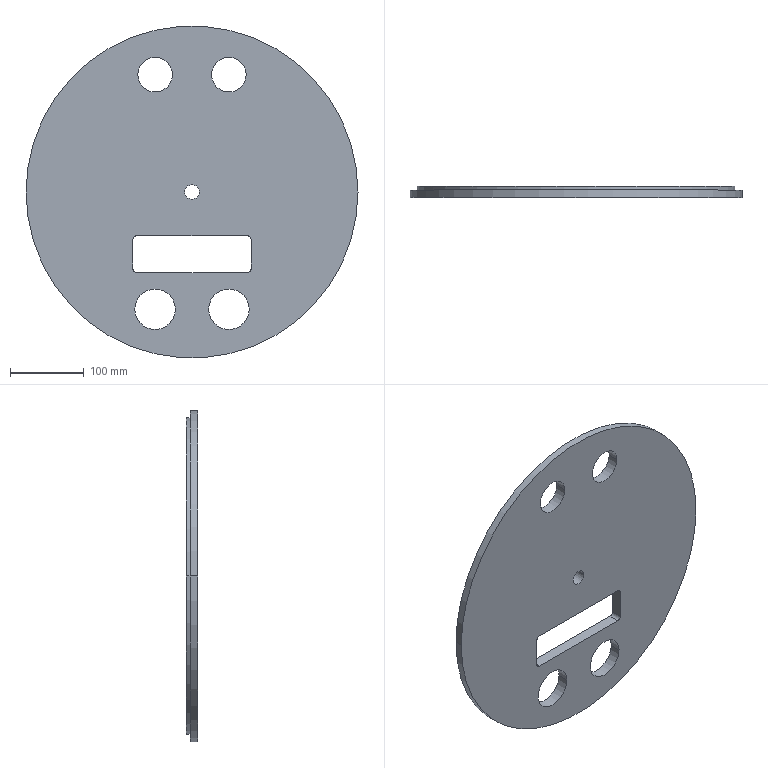Component | SolidWorks | Disc-1 | 1 solid | 25 faces | box 450 x 15 x 450 mm | volume 2068818 mm3 | cylinder 18 | plane 7 | commonest cylinder face diameters 47 x4 55 x4 10 x4 430 x2 20 x2 450 x2
build123d program:
from build123d import *

# Parameters (mm, degrees)
SKETCH1_R      = 225
EXTRUDE1_DEPTH = 15
SKETCH4_R      = 10
SKETCH4_R_2    = 27.5
SKETCH4_R_3    = 23.5
EXTRUDE3_DEPTH = 1808.804
EXTRUDE4_START = -5
SKETCH5_R      = 225
SKETCH5_R_2    = 215
EXTRUDE4_DEPTH = 5


with BuildPart() as part:
    # Sketch1 → Extrude1 (new body)
    with BuildSketch(Plane.XY):
        with Locations((1324.072, 706.83)):
            Circle(SKETCH1_R)
    extrude(amount=EXTRUDE1_DEPTH)

    # Sketch4 → Extrude3 (cut, through all)
    with BuildSketch(Plane(origin=(0, 0, 0), x_dir=(-1, 0, 0), z_dir=(0, 0, -1))):
        with Locations((-1324.072, 706.83)):
            Circle(SKETCH4_R)
        with Locations((-1374.072, 865.83)):
            Circle(SKETCH4_R_2)
        with Locations((-1274.072, 865.83)):
            Circle(SKETCH4_R_2)
        with Locations((-1374.072, 547.83)):
            Circle(SKETCH4_R_3)
        with Locations((-1274.072, 547.83)):
            Circle(SKETCH4_R_3)
        with BuildLine():
            Line((-1399.072, 766.33), (-1249.072, 766.33))
            ThreePointArc((-1249.072, 766.33), (-1245.536, 767.795), (-1244.072, 771.33))
            Line((-1244.072, 771.33), (-1244.072, 811.33))
            ThreePointArc((-1244.072, 811.33), (-1245.536, 814.866), (-1249.072, 816.33))
            Line((-1249.072, 816.33), (-1399.072, 816.33))
            ThreePointArc((-1399.072, 816.33), (-1402.607, 814.866), (-1404.072, 811.33))
            Line((-1404.072, 811.33), (-1404.072, 771.33))
            ThreePointArc((-1404.072, 771.33), (-1402.607, 767.795), (-1399.072, 766.33))
        make_face()
    extrude(amount=-EXTRUDE3_DEPTH, mode=Mode.SUBTRACT)

    # Sketch5 → Extrude4 (cut)
    with BuildSketch(Plane.XY.offset(15).offset(EXTRUDE4_START)):
        with Locations((1324.072, 706.83)):
            Circle(SKETCH5_R)
        with Locations((1324.072, 706.83)):
            Circle(SKETCH5_R_2, mode=Mode.SUBTRACT)
    extrude(amount=EXTRUDE4_DEPTH, mode=Mode.SUBTRACT)


solid = part.part

# Placed as in the assembly
solid = solid.moved(Location((-1488.855, 430.983, 710.83), (-90, 0, 0)))
STEP:
#1=COLOUR_RGB('',0.7922,0.8196,0.9333);
#2=FILL_AREA_STYLE_COLOUR('',#1);
#3=FILL_AREA_STYLE('',(#2));
#4=SURFACE_STYLE_FILL_AREA(#3);
#5=SURFACE_SIDE_STYLE('',(#4));
#6=SURFACE_STYLE_USAGE(.BOTH.,#5);
#7=PRESENTATION_STYLE_ASSIGNMENT((#6));
#8=CARTESIAN_POINT('',(1.977,17.362,0.1575));
#9=VERTEX_POINT('',#8);
#10=CARTESIAN_POINT('',(-14.952,17.362,0.1575));
#11=VERTEX_POINT('',#10);
#12=CARTESIAN_POINT('',(-6.488,17.362,0.1575));
#13=DIRECTION('',(0.,1.,0.));
#14=DIRECTION('',(1.,0.,-0.));
#15=AXIS2_PLACEMENT_3D('',#12,#13,#14);
#16=CIRCLE('',#15,8.465);
#17=EDGE_CURVE('',#9,#11,#16,.T.);
#18=ORIENTED_EDGE('',*,*,#17,.T.);
#19=CARTESIAN_POINT('',(-14.952,17.558,0.1575));
#20=VERTEX_POINT('',#19);
#21=CARTESIAN_POINT('',(-14.952,17.362,0.1575));
#22=DIRECTION('',(0.,1.,0.));
#23=VECTOR('',#22,39.37);
#24=LINE('',#21,#23);
#25=EDGE_CURVE('',#11,#20,#24,.T.);
#26=ORIENTED_EDGE('',*,*,#25,.T.);
#27=CARTESIAN_POINT('',(1.977,17.558,0.1575));
#28=VERTEX_POINT('',#27);
#29=CARTESIAN_POINT('',(-6.488,17.558,0.1575));
#30=DIRECTION('',(0.,1.,0.));
#31=DIRECTION('',(1.,0.,-0.));
#32=AXIS2_PLACEMENT_3D('',#29,#30,#31);
#33=CIRCLE('',#32,8.465);
#34=EDGE_CURVE('',#28,#20,#33,.T.);
#35=ORIENTED_EDGE('',*,*,#34,.F.);
#36=CARTESIAN_POINT('',(1.977,17.362,0.1575));
#37=DIRECTION('',(0.,1.,0.));
#38=VECTOR('',#37,39.37);
#39=LINE('',#36,#38);
#40=EDGE_CURVE('',#9,#28,#39,.T.);
#41=ORIENTED_EDGE('',*,*,#40,.F.);
#42=EDGE_LOOP('',(#18,#26,#35,#41));
#43=FACE_OUTER_BOUND('',#42,.T.);
#44=CARTESIAN_POINT('',(-6.488,17.362,0.1575));
#45=DIRECTION('',(0.,1.,0.));
#46=DIRECTION('',(1.,0.,-0.));
#47=AXIS2_PLACEMENT_3D('',#44,#45,#46);
#48=CYLINDRICAL_SURFACE('',#47,8.465);
#49=ADVANCED_FACE('',(#43),#48,.T.);
#50=CARTESIAN_POINT('',(-7.531,17.558,6.417));
#51=VERTEX_POINT('',#50);
#52=CARTESIAN_POINT('',(-9.381,17.558,6.417));
#53=VERTEX_POINT('',#52);
#54=CARTESIAN_POINT('',(-8.456,17.558,6.417));
#55=DIRECTION('',(0.,-1.,0.));
#56=DIRECTION('',(-1.,0.,0.));
#57=AXIS2_PLACEMENT_3D('',#54,#55,#56);
#58=CIRCLE('',#57,0.9252);
#59=EDGE_CURVE('',#51,#53,#58,.T.);
#60=ORIENTED_EDGE('',*,*,#59,.F.);
#61=CARTESIAN_POINT('',(-7.531,16.968,6.417));
#62=VERTEX_POINT('',#61);
#63=CARTESIAN_POINT('',(-7.531,17.558,6.417));
#64=DIRECTION('',(0.,-1.,0.));
#65=VECTOR('',#64,39.37);
#66=LINE('',#63,#65);
#67=EDGE_CURVE('',#51,#62,#66,.T.);
#68=ORIENTED_EDGE('',*,*,#67,.T.);
#69=CARTESIAN_POINT('',(-9.381,16.968,6.417));
#70=VERTEX_POINT('',#69);
#71=CARTESIAN_POINT('',(-8.456,16.968,6.417));
#72=DIRECTION('',(0.,-1.,0.));
#73=DIRECTION('',(-1.,0.,0.));
#74=AXIS2_PLACEMENT_3D('',#71,#72,#73);
#75=CIRCLE('',#74,0.9252);
#76=EDGE_CURVE('',#62,#70,#75,.T.);
#77=ORIENTED_EDGE('',*,*,#76,.T.);
#78=CARTESIAN_POINT('',(-9.381,17.558,6.417));
#79=DIRECTION('',(0.,-1.,0.));
#80=VECTOR('',#79,39.37);
#81=LINE('',#78,#80);
#82=EDGE_CURVE('',#53,#70,#81,.T.);
#83=ORIENTED_EDGE('',*,*,#82,.F.);
#84=EDGE_LOOP('',(#60,#68,#77,#83));
#85=FACE_OUTER_BOUND('',#84,.T.);
#86=CARTESIAN_POINT('',(-8.456,17.558,6.417));
#87=DIRECTION('',(0.,-1.,0.));
#88=DIRECTION('',(-1.,0.,0.));
#89=AXIS2_PLACEMENT_3D('',#86,#87,#88);
#90=CYLINDRICAL_SURFACE('',#89,0.9252);
#91=ADVANCED_FACE('',(#85),#90,.F.);
#92=CARTESIAN_POINT('',(-3.594,17.558,6.417));
#93=VERTEX_POINT('',#92);
#94=CARTESIAN_POINT('',(-5.444,17.558,6.417));
#95=VERTEX_POINT('',#94);
#96=CARTESIAN_POINT('',(-4.519,17.558,6.417));
#97=DIRECTION('',(0.,-1.,0.));
#98=DIRECTION('',(-1.,0.,0.));
#99=AXIS2_PLACEMENT_3D('',#96,#97,#98);
#100=CIRCLE('',#99,0.9252);
#101=EDGE_CURVE('',#93,#95,#100,.T.);
#102=ORIENTED_EDGE('',*,*,#101,.F.);
#103=CARTESIAN_POINT('',(-3.594,16.968,6.417));
#104=VERTEX_POINT('',#103);
#105=CARTESIAN_POINT('',(-3.594,17.558,6.417));
#106=DIRECTION('',(0.,-1.,0.));
#107=VECTOR('',#106,39.37);
#108=LINE('',#105,#107);
#109=EDGE_CURVE('',#93,#104,#108,.T.);
#110=ORIENTED_EDGE('',*,*,#109,.T.);
#111=CARTESIAN_POINT('',(-5.444,16.968,6.417));
#112=VERTEX_POINT('',#111);
#113=CARTESIAN_POINT('',(-4.519,16.968,6.417));
#114=DIRECTION('',(0.,-1.,0.));
#115=DIRECTION('',(-1.,0.,0.));
#116=AXIS2_PLACEMENT_3D('',#113,#114,#115);
#117=CIRCLE('',#116,0.9252);
#118=EDGE_CURVE('',#104,#112,#117,.T.);
#119=ORIENTED_EDGE('',*,*,#118,.T.);
#120=CARTESIAN_POINT('',(-5.444,17.558,6.417));
#121=DIRECTION('',(0.,-1.,0.));
#122=VECTOR('',#121,39.37);
#123=LINE('',#120,#122);
#124=EDGE_CURVE('',#95,#112,#123,.T.);
#125=ORIENTED_EDGE('',*,*,#124,.F.);
#126=EDGE_LOOP('',(#102,#110,#119,#125));
#127=FACE_OUTER_BOUND('',#126,.T.);
#128=CARTESIAN_POINT('',(-4.519,17.558,6.417));
#129=DIRECTION('',(0.,-1.,0.));
#130=DIRECTION('',(-1.,0.,0.));
#131=AXIS2_PLACEMENT_3D('',#128,#129,#130);
#132=CYLINDRICAL_SURFACE('',#131,0.9252);
#133=ADVANCED_FACE('',(#127),#132,.F.);
#134=CARTESIAN_POINT('',(-7.373,17.558,-6.102));
#135=VERTEX_POINT('',#134);
#136=CARTESIAN_POINT('',(-9.539,17.558,-6.102));
#137=VERTEX_POINT('',#136);
#138=CARTESIAN_POINT('',(-8.456,17.558,-6.102));
#139=DIRECTION('',(0.,-1.,0.));
#140=DIRECTION('',(-1.,0.,0.));
#141=AXIS2_PLACEMENT_3D('',#138,#139,#140);
#142=CIRCLE('',#141,1.083);
#143=EDGE_CURVE('',#135,#137,#142,.T.);
#144=ORIENTED_EDGE('',*,*,#143,.F.);
#145=CARTESIAN_POINT('',(-7.373,16.968,-6.102));
#146=VERTEX_POINT('',#145);
#147=CARTESIAN_POINT('',(-7.373,17.558,-6.102));
#148=DIRECTION('',(0.,-1.,0.));
#149=VECTOR('',#148,39.37);
#150=LINE('',#147,#149);
#151=EDGE_CURVE('',#135,#146,#150,.T.);
#152=ORIENTED_EDGE('',*,*,#151,.T.);
#153=CARTESIAN_POINT('',(-9.539,16.968,-6.102));
#154=VERTEX_POINT('',#153);
#155=CARTESIAN_POINT('',(-8.456,16.968,-6.102));
#156=DIRECTION('',(0.,-1.,0.));
#157=DIRECTION('',(-1.,0.,0.));
#158=AXIS2_PLACEMENT_3D('',#155,#156,#157);
#159=CIRCLE('',#158,1.083);
#160=EDGE_CURVE('',#146,#154,#159,.T.);
#161=ORIENTED_EDGE('',*,*,#160,.T.);
#162=CARTESIAN_POINT('',(-9.539,17.558,-6.102));
#163=DIRECTION('',(0.,-1.,0.));
#164=VECTOR('',#163,39.37);
#165=LINE('',#162,#164);
#166=EDGE_CURVE('',#137,#154,#165,.T.);
#167=ORIENTED_EDGE('',*,*,#166,.F.);
#168=EDGE_LOOP('',(#144,#152,#161,#167));
#169=FACE_OUTER_BOUND('',#168,.T.);
#170=CARTESIAN_POINT('',(-8.456,17.558,-6.102));
#171=DIRECTION('',(0.,-1.,0.));
#172=DIRECTION('',(-1.,0.,0.));
#173=AXIS2_PLACEMENT_3D('',#170,#171,#172);
#174=CYLINDRICAL_SURFACE('',#173,1.083);
#175=ADVANCED_FACE('',(#169),#174,.F.);
#176=CARTESIAN_POINT('',(-3.436,17.558,-6.102));
#177=VERTEX_POINT('',#176);
#178=CARTESIAN_POINT('',(-5.602,17.558,-6.102));
#179=VERTEX_POINT('',#178);
#180=CARTESIAN_POINT('',(-4.519,17.558,-6.102));
#181=DIRECTION('',(0.,-1.,0.));
#182=DIRECTION('',(-1.,0.,0.));
#183=AXIS2_PLACEMENT_3D('',#180,#181,#182);
#184=CIRCLE('',#183,1.083);
#185=EDGE_CURVE('',#177,#179,#184,.T.);
#186=ORIENTED_EDGE('',*,*,#185,.F.);
#187=CARTESIAN_POINT('',(-3.436,16.968,-6.102));
#188=VERTEX_POINT('',#187);
#189=CARTESIAN_POINT('',(-3.436,17.558,-6.102));
#190=DIRECTION('',(0.,-1.,0.));
#191=VECTOR('',#190,39.37);
#192=LINE('',#189,#191);
#193=EDGE_CURVE('',#177,#188,#192,.T.);
#194=ORIENTED_EDGE('',*,*,#193,.T.);
#195=CARTESIAN_POINT('',(-5.602,16.968,-6.102));
#196=VERTEX_POINT('',#195);
#197=CARTESIAN_POINT('',(-4.519,16.968,-6.102));
#198=DIRECTION('',(0.,-1.,0.));
#199=DIRECTION('',(-1.,0.,0.));
#200=AXIS2_PLACEMENT_3D('',#197,#198,#199);
#201=CIRCLE('',#200,1.083);
#202=EDGE_CURVE('',#188,#196,#201,.T.);
#203=ORIENTED_EDGE('',*,*,#202,.T.);
#204=CARTESIAN_POINT('',(-5.602,17.558,-6.102));
#205=DIRECTION('',(0.,-1.,0.));
#206=VECTOR('',#205,39.37);
#207=LINE('',#204,#206);
#208=EDGE_CURVE('',#179,#196,#207,.T.);
#209=ORIENTED_EDGE('',*,*,#208,.F.);
#210=EDGE_LOOP('',(#186,#194,#203,#209));
#211=FACE_OUTER_BOUND('',#210,.T.);
#212=CARTESIAN_POINT('',(-4.519,17.558,-6.102));
#213=DIRECTION('',(0.,-1.,0.));
#214=DIRECTION('',(-1.,0.,0.));
#215=AXIS2_PLACEMENT_3D('',#212,#213,#214);
#216=CYLINDRICAL_SURFACE('',#215,1.083);
#217=ADVANCED_FACE('',(#211),#216,.F.);
#218=CARTESIAN_POINT('',(-6.094,17.558,0.1575));
#219=VERTEX_POINT('',#218);
#220=CARTESIAN_POINT('',(-6.881,17.558,0.1575));
#221=VERTEX_POINT('',#220);
#222=CARTESIAN_POINT('',(-6.488,17.558,0.1575));
#223=DIRECTION('',(0.,-1.,0.));
#224=DIRECTION('',(-1.,0.,0.));
#225=AXIS2_PLACEMENT_3D('',#222,#223,#224);
#226=CIRCLE('',#225,0.3937);
#227=EDGE_CURVE('',#219,#221,#226,.T.);
#228=ORIENTED_EDGE('',*,*,#227,.F.);
#229=CARTESIAN_POINT('',(-6.094,16.968,0.1575));
#230=VERTEX_POINT('',#229);
#231=CARTESIAN_POINT('',(-6.094,17.558,0.1575));
#232=DIRECTION('',(0.,-1.,0.));
#233=VECTOR('',#232,39.37);
#234=LINE('',#231,#233);
#235=EDGE_CURVE('',#219,#230,#234,.T.);
#236=ORIENTED_EDGE('',*,*,#235,.T.);
#237=CARTESIAN_POINT('',(-6.881,16.968,0.1575));
#238=VERTEX_POINT('',#237);
#239=CARTESIAN_POINT('',(-6.488,16.968,0.1575));
#240=DIRECTION('',(0.,-1.,0.));
#241=DIRECTION('',(-1.,0.,0.));
#242=AXIS2_PLACEMENT_3D('',#239,#240,#241);
#243=CIRCLE('',#242,0.3937);
#244=EDGE_CURVE('',#230,#238,#243,.T.);
#245=ORIENTED_EDGE('',*,*,#244,.T.);
#246=CARTESIAN_POINT('',(-6.881,17.558,0.1575));
#247=DIRECTION('',(0.,-1.,0.));
#248=VECTOR('',#247,39.37);
#249=LINE('',#246,#248);
#250=EDGE_CURVE('',#221,#238,#249,.T.);
#251=ORIENTED_EDGE('',*,*,#250,.F.);
#252=EDGE_LOOP('',(#228,#236,#245,#251));
#253=FACE_OUTER_BOUND('',#252,.T.);
#254=CARTESIAN_POINT('',(-6.488,17.558,0.1575));
#255=DIRECTION('',(0.,-1.,0.));
#256=DIRECTION('',(-1.,0.,0.));
#257=AXIS2_PLACEMENT_3D('',#254,#255,#256);
#258=CYLINDRICAL_SURFACE('',#257,0.3937);
#259=ADVANCED_FACE('',(#253),#258,.F.);
#260=CARTESIAN_POINT('',(2.371,17.362,0.1575));
#261=VERTEX_POINT('',#260);
#262=CARTESIAN_POINT('',(-15.346,17.362,0.1575));
#263=VERTEX_POINT('',#262);
#264=CARTESIAN_POINT('',(-6.488,17.362,0.1575));
#265=DIRECTION('',(0.,1.,0.));
#266=DIRECTION('',(1.,0.,-0.));
#267=AXIS2_PLACEMENT_3D('',#264,#265,#266);
#268=CIRCLE('',#267,8.858);
#269=EDGE_CURVE('',#261,#263,#268,.T.);
#270=ORIENTED_EDGE('',*,*,#269,.F.);
#271=CARTESIAN_POINT('',(2.371,16.968,0.1575));
#272=VERTEX_POINT('',#271);
#273=CARTESIAN_POINT('',(2.371,17.558,0.1575));
#274=DIRECTION('',(0.,-1.,0.));
#275=VECTOR('',#274,39.37);
#276=LINE('',#273,#275);
#277=EDGE_CURVE('',#261,#272,#276,.T.);
#278=ORIENTED_EDGE('',*,*,#277,.T.);
#279=CARTESIAN_POINT('',(-15.346,16.968,0.1575));
#280=VERTEX_POINT('',#279);
#281=CARTESIAN_POINT('',(-6.488,16.968,0.1575));
#282=DIRECTION('',(0.,1.,0.));
#283=DIRECTION('',(1.,0.,-0.));
#284=AXIS2_PLACEMENT_3D('',#281,#282,#283);
#285=CIRCLE('',#284,8.858);
#286=EDGE_CURVE('',#272,#280,#285,.T.);
#287=ORIENTED_EDGE('',*,*,#286,.T.);
#288=CARTESIAN_POINT('',(-15.346,17.558,0.1575));
#289=DIRECTION('',(0.,-1.,0.));
#290=VECTOR('',#289,39.37);
#291=LINE('',#288,#290);
#292=EDGE_CURVE('',#263,#280,#291,.T.);
#293=ORIENTED_EDGE('',*,*,#292,.F.);
#294=EDGE_LOOP('',(#270,#278,#287,#293));
#295=FACE_OUTER_BOUND('',#294,.T.);
#296=CARTESIAN_POINT('',(-6.488,17.558,0.1575));
#297=DIRECTION('',(0.,-1.,0.));
#298=DIRECTION('',(-1.,0.,0.));
#299=AXIS2_PLACEMENT_3D('',#296,#297,#298);
#300=CYLINDRICAL_SURFACE('',#299,8.858);
#301=ADVANCED_FACE('',(#295),#300,.T.);
#302=ORIENTED_EDGE('',*,*,#277,.F.);
#303=CARTESIAN_POINT('',(-6.488,17.362,0.1575));
#304=DIRECTION('',(0.,1.,0.));
#305=DIRECTION('',(1.,0.,-0.));
#306=AXIS2_PLACEMENT_3D('',#303,#304,#305);
#307=CIRCLE('',#306,8.858);
#308=EDGE_CURVE('',#263,#261,#307,.T.);
#309=ORIENTED_EDGE('',*,*,#308,.F.);
#310=ORIENTED_EDGE('',*,*,#292,.T.);
#311=CARTESIAN_POINT('',(-6.488,16.968,0.1575));
#312=DIRECTION('',(0.,1.,0.));
#313=DIRECTION('',(1.,0.,-0.));
#314=AXIS2_PLACEMENT_3D('',#311,#312,#313);
#315=CIRCLE('',#314,8.858);
#316=EDGE_CURVE('',#280,#272,#315,.T.);
#317=ORIENTED_EDGE('',*,*,#316,.T.);
#318=EDGE_LOOP('',(#302,#309,#310,#317));
#319=FACE_OUTER_BOUND('',#318,.T.);
#320=CARTESIAN_POINT('',(-6.488,17.558,0.1575));
#321=DIRECTION('',(0.,-1.,0.));
#322=DIRECTION('',(-1.,0.,0.));
#323=AXIS2_PLACEMENT_3D('',#320,#321,#322);
#324=CYLINDRICAL_SURFACE('',#323,8.858);
#325=ADVANCED_FACE('',(#319),#324,.T.);
#326=CARTESIAN_POINT('',(-6.488,17.558,0.1575));
#327=DIRECTION('',(0.,-1.,0.));
#328=DIRECTION('',(-1.,0.,0.));
#329=AXIS2_PLACEMENT_3D('',#326,#327,#328);
#330=CIRCLE('',#329,0.3937);
#331=EDGE_CURVE('',#221,#219,#330,.T.);
#332=ORIENTED_EDGE('',*,*,#331,.T.);
#333=ORIENTED_EDGE('',*,*,#227,.T.);
#334=EDGE_LOOP('',(#332,#333));
#335=FACE_BOUND('',#334,.T.);
#336=CARTESIAN_POINT('',(-4.519,17.558,-6.102));
#337=DIRECTION('',(0.,-1.,0.));
#338=DIRECTION('',(-1.,0.,0.));
#339=AXIS2_PLACEMENT_3D('',#336,#337,#338);
#340=CIRCLE('',#339,1.083);
#341=EDGE_CURVE('',#179,#177,#340,.T.);
#342=ORIENTED_EDGE('',*,*,#341,.T.);
#343=ORIENTED_EDGE('',*,*,#185,.T.);
#344=EDGE_LOOP('',(#342,#343));
#345=FACE_BOUND('',#344,.T.);
#346=CARTESIAN_POINT('',(-8.456,17.558,-6.102));
#347=DIRECTION('',(0.,-1.,0.));
#348=DIRECTION('',(-1.,0.,0.));
#349=AXIS2_PLACEMENT_3D('',#346,#347,#348);
#350=CIRCLE('',#349,1.083);
#351=EDGE_CURVE('',#137,#135,#350,.T.);
#352=ORIENTED_EDGE('',*,*,#351,.T.);
#353=ORIENTED_EDGE('',*,*,#143,.T.);
#354=EDGE_LOOP('',(#352,#353));
#355=FACE_BOUND('',#354,.T.);
#356=CARTESIAN_POINT('',(-3.338,17.558,-2.382));
#357=VERTEX_POINT('',#356);
#358=CARTESIAN_POINT('',(-3.535,17.558,-2.185));
#359=VERTEX_POINT('',#358);
#360=CARTESIAN_POINT('',(-3.535,17.558,-2.382));
#361=DIRECTION('',(0.,-1.,0.));
#362=DIRECTION('',(-1.,0.,0.));
#363=AXIS2_PLACEMENT_3D('',#360,#361,#362);
#364=CIRCLE('',#363,0.1969);
#365=EDGE_CURVE('',#357,#359,#364,.T.);
#366=ORIENTED_EDGE('',*,*,#365,.T.);
#367=CARTESIAN_POINT('',(-9.44,17.558,-2.185));
#368=VERTEX_POINT('',#367);
#369=CARTESIAN_POINT('',(-3.535,17.558,-2.185));
#370=DIRECTION('',(-1.,0.,0.));
#371=VECTOR('',#370,39.37);
#372=LINE('',#369,#371);
#373=EDGE_CURVE('',#359,#368,#372,.T.);
#374=ORIENTED_EDGE('',*,*,#373,.T.);
#375=CARTESIAN_POINT('',(-9.637,17.558,-2.382));
#376=VERTEX_POINT('',#375);
#377=CARTESIAN_POINT('',(-9.44,17.558,-2.382));
#378=DIRECTION('',(0.,-1.,0.));
#379=DIRECTION('',(-1.,0.,0.));
#380=AXIS2_PLACEMENT_3D('',#377,#378,#379);
#381=CIRCLE('',#380,0.1969);
#382=EDGE_CURVE('',#368,#376,#381,.T.);
#383=ORIENTED_EDGE('',*,*,#382,.T.);
#384=CARTESIAN_POINT('',(-9.637,17.558,-3.957));
#385=VERTEX_POINT('',#384);
#386=CARTESIAN_POINT('',(-9.637,17.558,-2.382));
#387=DIRECTION('',(-0.,0.,-1.));
#388=VECTOR('',#387,39.37);
#389=LINE('',#386,#388);
#390=EDGE_CURVE('',#376,#385,#389,.T.);
#391=ORIENTED_EDGE('',*,*,#390,.T.);
#392=CARTESIAN_POINT('',(-9.44,17.558,-4.154));
#393=VERTEX_POINT('',#392);
#394=CARTESIAN_POINT('',(-9.44,17.558,-3.957));
#395=DIRECTION('',(0.,-1.,0.));
#396=DIRECTION('',(-1.,0.,0.));
#397=AXIS2_PLACEMENT_3D('',#394,#395,#396);
#398=CIRCLE('',#397,0.1969);
#399=EDGE_CURVE('',#385,#393,#398,.T.);
#400=ORIENTED_EDGE('',*,*,#399,.T.);
#401=CARTESIAN_POINT('',(-3.535,17.558,-4.154));
#402=VERTEX_POINT('',#401);
#403=CARTESIAN_POINT('',(-9.44,17.558,-4.154));
#404=DIRECTION('',(1.,0.,-0.));
#405=VECTOR('',#404,39.37);
#406=LINE('',#403,#405);
#407=EDGE_CURVE('',#393,#402,#406,.T.);
#408=ORIENTED_EDGE('',*,*,#407,.T.);
#409=CARTESIAN_POINT('',(-3.338,17.558,-3.957));
#410=VERTEX_POINT('',#409);
#411=CARTESIAN_POINT('',(-3.535,17.558,-3.957));
#412=DIRECTION('',(0.,-1.,0.));
#413=DIRECTION('',(-1.,0.,0.));
#414=AXIS2_PLACEMENT_3D('',#411,#412,#413);
#415=CIRCLE('',#414,0.1969);
#416=EDGE_CURVE('',#402,#410,#415,.T.);
#417=ORIENTED_EDGE('',*,*,#416,.T.);
#418=CARTESIAN_POINT('',(-3.338,17.558,-3.957));
#419=DIRECTION('',(0.,0.,1.));
#420=VECTOR('',#419,39.37);
#421=LINE('',#418,#420);
#422=EDGE_CURVE('',#410,#357,#421,.T.);
#423=ORIENTED_EDGE('',*,*,#422,.T.);
#424=EDGE_LOOP('',(#366,#374,#383,#391,#400,#408,#417,#423));
#425=FACE_BOUND('',#424,.T.);
#426=CARTESIAN_POINT('',(-4.519,17.558,6.417));
#427=DIRECTION('',(0.,-1.,0.));
#428=DIRECTION('',(-1.,0.,0.));
#429=AXIS2_PLACEMENT_3D('',#426,#427,#428);
#430=CIRCLE('',#429,0.9252);
#431=EDGE_CURVE('',#95,#93,#430,.T.);
#432=ORIENTED_EDGE('',*,*,#431,.T.);
#433=ORIENTED_EDGE('',*,*,#101,.T.);
#434=EDGE_LOOP('',(#432,#433));
#435=FACE_BOUND('',#434,.T.);
#436=CARTESIAN_POINT('',(-8.456,17.558,6.417));
#437=DIRECTION('',(0.,-1.,0.));
#438=DIRECTION('',(-1.,0.,0.));
#439=AXIS2_PLACEMENT_3D('',#436,#437,#438);
#440=CIRCLE('',#439,0.9252);
#441=EDGE_CURVE('',#53,#51,#440,.T.);
#442=ORIENTED_EDGE('',*,*,#441,.T.);
#443=ORIENTED_EDGE('',*,*,#59,.T.);
#444=EDGE_LOOP('',(#442,#443));
#445=FACE_BOUND('',#444,.T.);
#446=ORIENTED_EDGE('',*,*,#34,.T.);
#447=CARTESIAN_POINT('',(-6.488,17.558,0.1575));
#448=DIRECTION('',(0.,1.,0.));
#449=DIRECTION('',(1.,0.,-0.));
#450=AXIS2_PLACEMENT_3D('',#447,#448,#449);
#451=CIRCLE('',#450,8.465);
#452=EDGE_CURVE('',#20,#28,#451,.T.);
#453=ORIENTED_EDGE('',*,*,#452,.T.);
#454=EDGE_LOOP('',(#446,#453));
#455=FACE_OUTER_BOUND('',#454,.T.);
#456=CARTESIAN_POINT('',(-6.488,17.558,0.1575));
#457=DIRECTION('',(0.,1.,0.));
#458=DIRECTION('',(1.,0.,-0.));
#459=AXIS2_PLACEMENT_3D('',#456,#457,#458);
#460=PLANE('',#459);
#461=ADVANCED_FACE('',(#335,#345,#355,#425,#435,#445,#455),#460,.T.);
#462=CARTESIAN_POINT('',(-8.456,16.968,6.417));
#463=DIRECTION('',(0.,-1.,0.));
#464=DIRECTION('',(-1.,0.,0.));
#465=AXIS2_PLACEMENT_3D('',#462,#463,#464);
#466=CIRCLE('',#465,0.9252);
#467=EDGE_CURVE('',#70,#62,#466,.T.);
#468=ORIENTED_EDGE('',*,*,#467,.F.);
#469=ORIENTED_EDGE('',*,*,#76,.F.);
#470=EDGE_LOOP('',(#468,#469));
#471=FACE_BOUND('',#470,.T.);
#472=CARTESIAN_POINT('',(-4.519,16.968,6.417));
#473=DIRECTION('',(0.,-1.,0.));
#474=DIRECTION('',(-1.,0.,0.));
#475=AXIS2_PLACEMENT_3D('',#472,#473,#474);
#476=CIRCLE('',#475,0.9252);
#477=EDGE_CURVE('',#112,#104,#476,.T.);
#478=ORIENTED_EDGE('',*,*,#477,.F.);
#479=ORIENTED_EDGE('',*,*,#118,.F.);
#480=EDGE_LOOP('',(#478,#479));
#481=FACE_BOUND('',#480,.T.);
#482=CARTESIAN_POINT('',(-3.535,16.968,-2.185));
#483=VERTEX_POINT('',#482);
#484=CARTESIAN_POINT('',(-9.44,16.968,-2.185));
#485=VERTEX_POINT('',#484);
#486=CARTESIAN_POINT('',(-3.535,16.968,-2.185));
#487=DIRECTION('',(-1.,0.,0.));
#488=VECTOR('',#487,39.37);
#489=LINE('',#486,#488);
#490=EDGE_CURVE('',#483,#485,#489,.T.);
#491=ORIENTED_EDGE('',*,*,#490,.F.);
#492=CARTESIAN_POINT('',(-3.338,16.968,-2.382));
#493=VERTEX_POINT('',#492);
#494=CARTESIAN_POINT('',(-3.535,16.968,-2.382));
#495=DIRECTION('',(0.,-1.,0.));
#496=DIRECTION('',(-1.,0.,0.));
#497=AXIS2_PLACEMENT_3D('',#494,#495,#496);
#498=CIRCLE('',#497,0.1969);
#499=EDGE_CURVE('',#493,#483,#498,.T.);
#500=ORIENTED_EDGE('',*,*,#499,.F.);
#501=CARTESIAN_POINT('',(-3.338,16.968,-3.957));
#502=VERTEX_POINT('',#501);
#503=CARTESIAN_POINT('',(-3.338,16.968,-3.957));
#504=DIRECTION('',(0.,0.,1.));
#505=VECTOR('',#504,39.37);
#506=LINE('',#503,#505);
#507=EDGE_CURVE('',#502,#493,#506,.T.);
#508=ORIENTED_EDGE('',*,*,#507,.F.);
#509=CARTESIAN_POINT('',(-3.535,16.968,-4.154));
#510=VERTEX_POINT('',#509);
#511=CARTESIAN_POINT('',(-3.535,16.968,-3.957));
#512=DIRECTION('',(0.,-1.,0.));
#513=DIRECTION('',(-1.,0.,0.));
#514=AXIS2_PLACEMENT_3D('',#511,#512,#513);
#515=CIRCLE('',#514,0.1969);
#516=EDGE_CURVE('',#510,#502,#515,.T.);
#517=ORIENTED_EDGE('',*,*,#516,.F.);
#518=CARTESIAN_POINT('',(-9.44,16.968,-4.154));
#519=VERTEX_POINT('',#518);
#520=CARTESIAN_POINT('',(-9.44,16.968,-4.154));
#521=DIRECTION('',(1.,0.,-0.));
#522=VECTOR('',#521,39.37);
#523=LINE('',#520,#522);
#524=EDGE_CURVE('',#519,#510,#523,.T.);
#525=ORIENTED_EDGE('',*,*,#524,.F.);
#526=CARTESIAN_POINT('',(-9.637,16.968,-3.957));
#527=VERTEX_POINT('',#526);
#528=CARTESIAN_POINT('',(-9.44,16.968,-3.957));
#529=DIRECTION('',(0.,-1.,0.));
#530=DIRECTION('',(-1.,0.,0.));
#531=AXIS2_PLACEMENT_3D('',#528,#529,#530);
#532=CIRCLE('',#531,0.1969);
#533=EDGE_CURVE('',#527,#519,#532,.T.);
#534=ORIENTED_EDGE('',*,*,#533,.F.);
#535=CARTESIAN_POINT('',(-9.637,16.968,-2.382));
#536=VERTEX_POINT('',#535);
#537=CARTESIAN_POINT('',(-9.637,16.968,-2.382));
#538=DIRECTION('',(-0.,0.,-1.));
#539=VECTOR('',#538,39.37);
#540=LINE('',#537,#539);
#541=EDGE_CURVE('',#536,#527,#540,.T.);
#542=ORIENTED_EDGE('',*,*,#541,.F.);
#543=CARTESIAN_POINT('',(-9.44,16.968,-2.382));
#544=DIRECTION('',(0.,-1.,0.));
#545=DIRECTION('',(-1.,0.,0.));
#546=AXIS2_PLACEMENT_3D('',#543,#544,#545);
#547=CIRCLE('',#546,0.1969);
#548=EDGE_CURVE('',#485,#536,#547,.T.);
#549=ORIENTED_EDGE('',*,*,#548,.F.);
#550=EDGE_LOOP('',(#491,#500,#508,#517,#525,#534,#542,#549));
#551=FACE_BOUND('',#550,.T.);
#552=CARTESIAN_POINT('',(-8.456,16.968,-6.102));
#553=DIRECTION('',(0.,-1.,0.));
#554=DIRECTION('',(-1.,0.,0.));
#555=AXIS2_PLACEMENT_3D('',#552,#553,#554);
#556=CIRCLE('',#555,1.083);
#557=EDGE_CURVE('',#154,#146,#556,.T.);
#558=ORIENTED_EDGE('',*,*,#557,.F.);
#559=ORIENTED_EDGE('',*,*,#160,.F.);
#560=EDGE_LOOP('',(#558,#559));
#561=FACE_BOUND('',#560,.T.);
#562=CARTESIAN_POINT('',(-4.519,16.968,-6.102));
#563=DIRECTION('',(0.,-1.,0.));
#564=DIRECTION('',(-1.,0.,0.));
#565=AXIS2_PLACEMENT_3D('',#562,#563,#564);
#566=CIRCLE('',#565,1.083);
#567=EDGE_CURVE('',#196,#188,#566,.T.);
#568=ORIENTED_EDGE('',*,*,#567,.F.);
#569=ORIENTED_EDGE('',*,*,#202,.F.);
#570=EDGE_LOOP('',(#568,#569));
#571=FACE_BOUND('',#570,.T.);
#572=CARTESIAN_POINT('',(-6.488,16.968,0.1575));
#573=DIRECTION('',(0.,-1.,0.));
#574=DIRECTION('',(-1.,0.,0.));
#575=AXIS2_PLACEMENT_3D('',#572,#573,#574);
#576=CIRCLE('',#575,0.3937);
#577=EDGE_CURVE('',#238,#230,#576,.T.);
#578=ORIENTED_EDGE('',*,*,#577,.F.);
#579=ORIENTED_EDGE('',*,*,#244,.F.);
#580=EDGE_LOOP('',(#578,#579));
#581=FACE_BOUND('',#580,.T.);
#582=ORIENTED_EDGE('',*,*,#316,.F.);
#583=ORIENTED_EDGE('',*,*,#286,.F.);
#584=EDGE_LOOP('',(#582,#583));
#585=FACE_OUTER_BOUND('',#584,.T.);
#586=CARTESIAN_POINT('',(-6.488,16.968,0.1575));
#587=DIRECTION('',(0.,1.,0.));
#588=DIRECTION('',(1.,0.,-0.));
#589=AXIS2_PLACEMENT_3D('',#586,#587,#588);
#590=PLANE('',#589);
#591=ADVANCED_FACE('',(#471,#481,#551,#561,#571,#581,#585),#590,.F.);
#592=ORIENTED_EDGE('',*,*,#235,.F.);
#593=ORIENTED_EDGE('',*,*,#331,.F.);
#594=ORIENTED_EDGE('',*,*,#250,.T.);
#595=ORIENTED_EDGE('',*,*,#577,.T.);
#596=EDGE_LOOP('',(#592,#593,#594,#595));
#597=FACE_OUTER_BOUND('',#596,.T.);
#598=CARTESIAN_POINT('',(-6.488,17.558,0.1575));
#599=DIRECTION('',(0.,-1.,0.));
#600=DIRECTION('',(-1.,0.,0.));
#601=AXIS2_PLACEMENT_3D('',#598,#599,#600);
#602=CYLINDRICAL_SURFACE('',#601,0.3937);
#603=ADVANCED_FACE('',(#597),#602,.F.);
#604=ORIENTED_EDGE('',*,*,#193,.F.);
#605=ORIENTED_EDGE('',*,*,#341,.F.);
#606=ORIENTED_EDGE('',*,*,#208,.T.);
#607=ORIENTED_EDGE('',*,*,#567,.T.);
#608=EDGE_LOOP('',(#604,#605,#606,#607));
#609=FACE_OUTER_BOUND('',#608,.T.);
#610=CARTESIAN_POINT('',(-4.519,17.558,-6.102));
#611=DIRECTION('',(0.,-1.,0.));
#612=DIRECTION('',(-1.,0.,0.));
#613=AXIS2_PLACEMENT_3D('',#610,#611,#612);
#614=CYLINDRICAL_SURFACE('',#613,1.083);
#615=ADVANCED_FACE('',(#609),#614,.F.);
#616=ORIENTED_EDGE('',*,*,#151,.F.);
#617=ORIENTED_EDGE('',*,*,#351,.F.);
#618=ORIENTED_EDGE('',*,*,#166,.T.);
#619=ORIENTED_EDGE('',*,*,#557,.T.);
#620=EDGE_LOOP('',(#616,#617,#618,#619));
#621=FACE_OUTER_BOUND('',#620,.T.);
#622=CARTESIAN_POINT('',(-8.456,17.558,-6.102));
#623=DIRECTION('',(0.,-1.,0.));
#624=DIRECTION('',(-1.,0.,0.));
#625=AXIS2_PLACEMENT_3D('',#622,#623,#624);
#626=CYLINDRICAL_SURFACE('',#625,1.083);
#627=ADVANCED_FACE('',(#621),#626,.F.);
#628=ORIENTED_EDGE('',*,*,#499,.T.);
#629=CARTESIAN_POINT('',(-3.535,17.558,-2.185));
#630=DIRECTION('',(0.,-1.,0.));
#631=VECTOR('',#630,39.37);
#632=LINE('',#629,#631);
#633=EDGE_CURVE('',#359,#483,#632,.T.);
#634=ORIENTED_EDGE('',*,*,#633,.F.);
#635=ORIENTED_EDGE('',*,*,#365,.F.);
#636=CARTESIAN_POINT('',(-3.338,17.558,-2.382));
#637=DIRECTION('',(0.,-1.,0.));
#638=VECTOR('',#637,39.37);
#639=LINE('',#636,#638);
#640=EDGE_CURVE('',#357,#493,#639,.T.);
#641=ORIENTED_EDGE('',*,*,#640,.T.);
#642=EDGE_LOOP('',(#628,#634,#635,#641));
#643=FACE_OUTER_BOUND('',#642,.T.);
#644=CARTESIAN_POINT('',(-3.535,17.558,-2.382));
#645=DIRECTION('',(0.,-1.,0.));
#646=DIRECTION('',(-1.,0.,0.));
#647=AXIS2_PLACEMENT_3D('',#644,#645,#646);
#648=CYLINDRICAL_SURFACE('',#647,0.1969);
#649=ADVANCED_FACE('',(#643),#648,.F.);
#650=ORIENTED_EDGE('',*,*,#507,.T.);
#651=ORIENTED_EDGE('',*,*,#640,.F.);
#652=ORIENTED_EDGE('',*,*,#422,.F.);
#653=CARTESIAN_POINT('',(-3.338,17.558,-3.957));
#654=DIRECTION('',(0.,-1.,0.));
#655=VECTOR('',#654,39.37);
#656=LINE('',#653,#655);
#657=EDGE_CURVE('',#410,#502,#656,.T.);
#658=ORIENTED_EDGE('',*,*,#657,.T.);
#659=EDGE_LOOP('',(#650,#651,#652,#658));
#660=FACE_OUTER_BOUND('',#659,.T.);
#661=CARTESIAN_POINT('',(-3.338,17.558,-3.957));
#662=DIRECTION('',(1.,0.,-0.));
#663=DIRECTION('',(-0.,0.,-1.));
#664=AXIS2_PLACEMENT_3D('',#661,#662,#663);
#665=PLANE('',#664);
#666=ADVANCED_FACE('',(#660),#665,.F.);
#667=ORIENTED_EDGE('',*,*,#516,.T.);
#668=ORIENTED_EDGE('',*,*,#657,.F.);
#669=ORIENTED_EDGE('',*,*,#416,.F.);
#670=CARTESIAN_POINT('',(-3.535,17.558,-4.154));
#671=DIRECTION('',(0.,-1.,0.));
#672=VECTOR('',#671,39.37);
#673=LINE('',#670,#672);
#674=EDGE_CURVE('',#402,#510,#673,.T.);
#675=ORIENTED_EDGE('',*,*,#674,.T.);
#676=EDGE_LOOP('',(#667,#668,#669,#675));
#677=FACE_OUTER_BOUND('',#676,.T.);
#678=CARTESIAN_POINT('',(-3.535,17.558,-3.957));
#679=DIRECTION('',(0.,-1.,0.));
#680=DIRECTION('',(-1.,0.,0.));
#681=AXIS2_PLACEMENT_3D('',#678,#679,#680);
#682=CYLINDRICAL_SURFACE('',#681,0.1969);
#683=ADVANCED_FACE('',(#677),#682,.F.);
#684=ORIENTED_EDGE('',*,*,#524,.T.);
#685=ORIENTED_EDGE('',*,*,#674,.F.);
#686=ORIENTED_EDGE('',*,*,#407,.F.);
#687=CARTESIAN_POINT('',(-9.44,17.558,-4.154));
#688=DIRECTION('',(0.,-1.,0.));
#689=VECTOR('',#688,39.37);
#690=LINE('',#687,#689);
#691=EDGE_CURVE('',#393,#519,#690,.T.);
#692=ORIENTED_EDGE('',*,*,#691,.T.);
#693=EDGE_LOOP('',(#684,#685,#686,#692));
#694=FACE_OUTER_BOUND('',#693,.T.);
#695=CARTESIAN_POINT('',(-9.44,17.558,-4.154));
#696=DIRECTION('',(-0.,0.,-1.));
#697=DIRECTION('',(-1.,0.,0.));
#698=AXIS2_PLACEMENT_3D('',#695,#696,#697);
#699=PLANE('',#698);
#700=ADVANCED_FACE('',(#694),#699,.F.);
#701=ORIENTED_EDGE('',*,*,#533,.T.);
#702=ORIENTED_EDGE('',*,*,#691,.F.);
#703=ORIENTED_EDGE('',*,*,#399,.F.);
#704=CARTESIAN_POINT('',(-9.637,17.558,-3.957));
#705=DIRECTION('',(0.,-1.,0.));
#706=VECTOR('',#705,39.37);
#707=LINE('',#704,#706);
#708=EDGE_CURVE('',#385,#527,#707,.T.);
#709=ORIENTED_EDGE('',*,*,#708,.T.);
#710=EDGE_LOOP('',(#701,#702,#703,#709));
#711=FACE_OUTER_BOUND('',#710,.T.);
#712=CARTESIAN_POINT('',(-9.44,17.558,-3.957));
#713=DIRECTION('',(0.,-1.,0.));
#714=DIRECTION('',(-1.,0.,0.));
#715=AXIS2_PLACEMENT_3D('',#712,#713,#714);
#716=CYLINDRICAL_SURFACE('',#715,0.1969);
#717=ADVANCED_FACE('',(#711),#716,.F.);
#718=ORIENTED_EDGE('',*,*,#541,.T.);
#719=ORIENTED_EDGE('',*,*,#708,.F.);
#720=ORIENTED_EDGE('',*,*,#390,.F.);
#721=CARTESIAN_POINT('',(-9.637,17.558,-2.382));
#722=DIRECTION('',(0.,-1.,0.));
#723=VECTOR('',#722,39.37);
#724=LINE('',#721,#723);
#725=EDGE_CURVE('',#376,#536,#724,.T.);
#726=ORIENTED_EDGE('',*,*,#725,.T.);
#727=EDGE_LOOP('',(#718,#719,#720,#726));
#728=FACE_OUTER_BOUND('',#727,.T.);
#729=CARTESIAN_POINT('',(-9.637,17.558,-2.382));
#730=DIRECTION('',(-1.,0.,0.));
#731=DIRECTION('',(0.,1.,0.));
#732=AXIS2_PLACEMENT_3D('',#729,#730,#731);
#733=PLANE('',#732);
#734=ADVANCED_FACE('',(#728),#733,.F.);
#735=ORIENTED_EDGE('',*,*,#548,.T.);
#736=ORIENTED_EDGE('',*,*,#725,.F.);
#737=ORIENTED_EDGE('',*,*,#382,.F.);
#738=CARTESIAN_POINT('',(-9.44,17.558,-2.185));
#739=DIRECTION('',(0.,-1.,0.));
#740=VECTOR('',#739,39.37);
#741=LINE('',#738,#740);
#742=EDGE_CURVE('',#368,#485,#741,.T.);
#743=ORIENTED_EDGE('',*,*,#742,.T.);
#744=EDGE_LOOP('',(#735,#736,#737,#743));
#745=FACE_OUTER_BOUND('',#744,.T.);
#746=CARTESIAN_POINT('',(-9.44,17.558,-2.382));
#747=DIRECTION('',(0.,-1.,0.));
#748=DIRECTION('',(-1.,0.,0.));
#749=AXIS2_PLACEMENT_3D('',#746,#747,#748);
#750=CYLINDRICAL_SURFACE('',#749,0.1969);
#751=ADVANCED_FACE('',(#745),#750,.F.);
#752=ORIENTED_EDGE('',*,*,#490,.T.);
#753=ORIENTED_EDGE('',*,*,#742,.F.);
#754=ORIENTED_EDGE('',*,*,#373,.F.);
#755=ORIENTED_EDGE('',*,*,#633,.T.);
#756=EDGE_LOOP('',(#752,#753,#754,#755));
#757=FACE_OUTER_BOUND('',#756,.T.);
#758=CARTESIAN_POINT('',(-3.535,17.558,-2.185));
#759=DIRECTION('',(0.,0.,1.));
#760=DIRECTION('',(0.,-1.,0.));
#761=AXIS2_PLACEMENT_3D('',#758,#759,#760);
#762=PLANE('',#761);
#763=ADVANCED_FACE('',(#757),#762,.F.);
#764=ORIENTED_EDGE('',*,*,#109,.F.);
#765=ORIENTED_EDGE('',*,*,#431,.F.);
#766=ORIENTED_EDGE('',*,*,#124,.T.);
#767=ORIENTED_EDGE('',*,*,#477,.T.);
#768=EDGE_LOOP('',(#764,#765,#766,#767));
#769=FACE_OUTER_BOUND('',#768,.T.);
#770=CARTESIAN_POINT('',(-4.519,17.558,6.417));
#771=DIRECTION('',(0.,-1.,0.));
#772=DIRECTION('',(-1.,0.,0.));
#773=AXIS2_PLACEMENT_3D('',#770,#771,#772);
#774=CYLINDRICAL_SURFACE('',#773,0.9252);
#775=ADVANCED_FACE('',(#769),#774,.F.);
#776=ORIENTED_EDGE('',*,*,#67,.F.);
#777=ORIENTED_EDGE('',*,*,#441,.F.);
#778=ORIENTED_EDGE('',*,*,#82,.T.);
#779=ORIENTED_EDGE('',*,*,#467,.T.);
#780=EDGE_LOOP('',(#776,#777,#778,#779));
#781=FACE_OUTER_BOUND('',#780,.T.);
#782=CARTESIAN_POINT('',(-8.456,17.558,6.417));
#783=DIRECTION('',(0.,-1.,0.));
#784=DIRECTION('',(-1.,0.,0.));
#785=AXIS2_PLACEMENT_3D('',#782,#783,#784);
#786=CYLINDRICAL_SURFACE('',#785,0.9252);
#787=ADVANCED_FACE('',(#781),#786,.F.);
#788=ORIENTED_EDGE('',*,*,#17,.F.);
#789=CARTESIAN_POINT('',(-6.488,17.362,0.1575));
#790=DIRECTION('',(0.,1.,0.));
#791=DIRECTION('',(1.,0.,-0.));
#792=AXIS2_PLACEMENT_3D('',#789,#790,#791);
#793=CIRCLE('',#792,8.465);
#794=EDGE_CURVE('',#11,#9,#793,.T.);
#795=ORIENTED_EDGE('',*,*,#794,.F.);
#796=EDGE_LOOP('',(#788,#795));
#797=FACE_BOUND('',#796,.T.);
#798=ORIENTED_EDGE('',*,*,#308,.T.);
#799=ORIENTED_EDGE('',*,*,#269,.T.);
#800=EDGE_LOOP('',(#798,#799));
#801=FACE_OUTER_BOUND('',#800,.T.);
#802=CARTESIAN_POINT('',(-6.488,17.362,0.1575));
#803=DIRECTION('',(0.,1.,0.));
#804=DIRECTION('',(1.,0.,-0.));
#805=AXIS2_PLACEMENT_3D('',#802,#803,#804);
#806=PLANE('',#805);
#807=ADVANCED_FACE('',(#797,#801),#806,.T.);
#808=ORIENTED_EDGE('',*,*,#25,.F.);
#809=ORIENTED_EDGE('',*,*,#794,.T.);
#810=ORIENTED_EDGE('',*,*,#40,.T.);
#811=ORIENTED_EDGE('',*,*,#452,.F.);
#812=EDGE_LOOP('',(#808,#809,#810,#811));
#813=FACE_OUTER_BOUND('',#812,.T.);
#814=CARTESIAN_POINT('',(-6.488,17.362,0.1575));
#815=DIRECTION('',(0.,1.,0.));
#816=DIRECTION('',(1.,0.,-0.));
#817=AXIS2_PLACEMENT_3D('',#814,#815,#816);
#818=CYLINDRICAL_SURFACE('',#817,8.465);
#819=ADVANCED_FACE('',(#813),#818,.T.);
#820=CLOSED_SHELL('',(#49,#91,#133,#175,#217,#259,#301,#325,#461,#591,#603,#615,#627,#649,#666,#683,#700,#717,#734,#751,#763,#775,#787,#807,#819));
#821=MANIFOLD_SOLID_BREP('',#820);
#822=STYLED_ITEM('',(#7),#821);
#823=(LENGTH_UNIT()NAMED_UNIT(*)SI_UNIT($,.METRE.));
#824=LENGTH_MEASURE_WITH_UNIT(LENGTH_MEASURE(0.0254),#823);
#825=DIMENSIONAL_EXPONENTS(1.,0.,0.,0.,0.,0.,0.);
#826=(CONVERSION_BASED_UNIT('',#824)LENGTH_UNIT()NAMED_UNIT(#825));
#827=UNCERTAINTY_MEASURE_WITH_UNIT(LENGTH_MEASURE(0.00001),#826,'','');
#828=(NAMED_UNIT(*)PLANE_ANGLE_UNIT()SI_UNIT($,.RADIAN.));
#829=(NAMED_UNIT(*)SI_UNIT($,.STERADIAN.)SOLID_ANGLE_UNIT());
#830=(GEOMETRIC_REPRESENTATION_CONTEXT(3)GLOBAL_UNCERTAINTY_ASSIGNED_CONTEXT((#827))GLOBAL_UNIT_ASSIGNED_CONTEXT((#826,#828,#829))REPRESENTATION_CONTEXT('',''));
#831=MECHANICAL_DESIGN_GEOMETRIC_PRESENTATION_REPRESENTATION('',(#822),#830);
#832=PRESENTATION_LAYER_ASSIGNMENT('','',(#822));
#833=CARTESIAN_POINT('',(0.,0.,0.));
#834=DIRECTION('',(0.,0.,1.));
#835=DIRECTION('',(1.,0.,0.));
#836=AXIS2_PLACEMENT_3D('',#833,#834,#835);
#837=(LENGTH_UNIT()NAMED_UNIT(*)SI_UNIT($,.METRE.));
#838=LENGTH_MEASURE_WITH_UNIT(LENGTH_MEASURE(0.0254),#837);
#839=DIMENSIONAL_EXPONENTS(1.,0.,0.,0.,0.,0.,0.);
#840=(CONVERSION_BASED_UNIT('',#838)LENGTH_UNIT()NAMED_UNIT(#839));
#841=UNCERTAINTY_MEASURE_WITH_UNIT(LENGTH_MEASURE(0.00001),#840,'','');
#842=(NAMED_UNIT(*)PLANE_ANGLE_UNIT()SI_UNIT($,.RADIAN.));
#843=(NAMED_UNIT(*)SI_UNIT($,.STERADIAN.)SOLID_ANGLE_UNIT());
#844=(GEOMETRIC_REPRESENTATION_CONTEXT(3)GLOBAL_UNCERTAINTY_ASSIGNED_CONTEXT((#841))GLOBAL_UNIT_ASSIGNED_CONTEXT((#840,#842,#843))REPRESENTATION_CONTEXT('',''));
#845=ADVANCED_BREP_SHAPE_REPRESENTATION('',(#821,#836),#844);